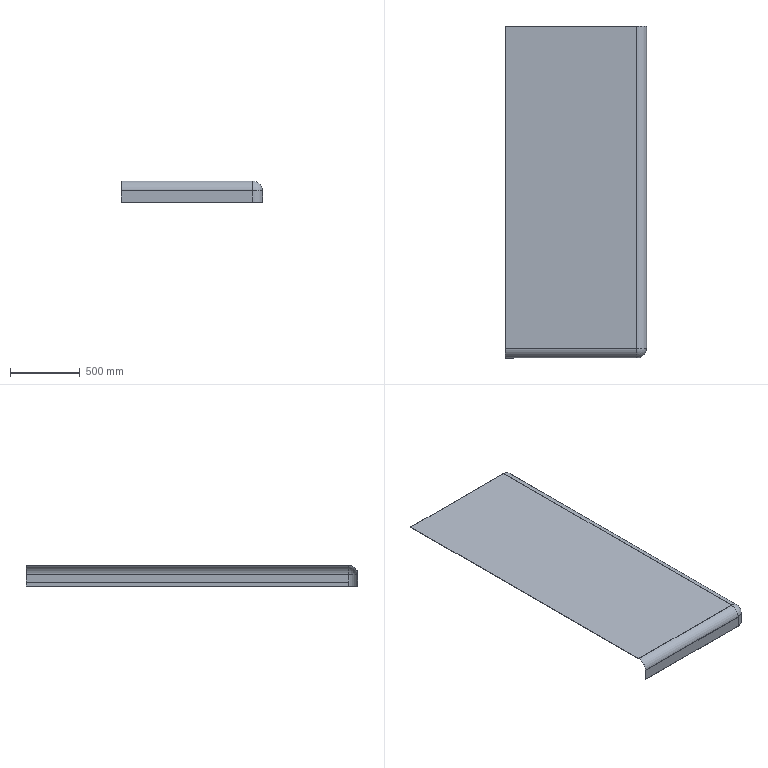Component | SolidWorks | A-SideAluminumCasingAssembly-1_A-SideAluminumCasing3-1 | 1 solid | 38 faces | box 1009.5 x 2375.5 x 154.5 mm | volume 8957048 mm3 | plane 26 | cylinder 10 | torus 2 | commonest cylinder face diameters 139 x2 133 x2 10 x2 4 x2 141 x1 135 x1
STEP:
#1=COLOUR_RGB('',0.7922,0.8196,0.9333);
#2=FILL_AREA_STYLE_COLOUR('',#1);
#3=FILL_AREA_STYLE('',(#2));
#4=SURFACE_STYLE_FILL_AREA(#3);
#5=SURFACE_SIDE_STYLE('',(#4));
#6=SURFACE_STYLE_USAGE(.BOTH.,#5);
#7=PRESENTATION_STYLE_ASSIGNMENT((#6));
#8=CARTESIAN_POINT('',(43.543,0.,73.937));
#9=VERTEX_POINT('',#8);
#10=CARTESIAN_POINT('',(43.543,0.,73.819));
#11=VERTEX_POINT('',#10);
#12=CARTESIAN_POINT('',(43.543,0.,73.819));
#13=DIRECTION('',(0.,-0.,-1.));
#14=VECTOR('',#13,39.37);
#15=LINE('',#12,#14);
#16=EDGE_CURVE('',#9,#11,#15,.T.);
#17=ORIENTED_EDGE('',*,*,#16,.F.);
#18=CARTESIAN_POINT('',(43.543,90.787,73.937));
#19=VERTEX_POINT('',#18);
#20=CARTESIAN_POINT('',(43.543,0.,73.937));
#21=DIRECTION('',(-0.,1.,-0.));
#22=VECTOR('',#21,39.37);
#23=LINE('',#20,#22);
#24=EDGE_CURVE('',#9,#19,#23,.T.);
#25=ORIENTED_EDGE('',*,*,#24,.T.);
#26=CARTESIAN_POINT('',(43.543,90.787,73.819));
#27=VERTEX_POINT('',#26);
#28=CARTESIAN_POINT('',(43.543,90.787,73.819));
#29=DIRECTION('',(0.,-0.,-1.));
#30=VECTOR('',#29,39.37);
#31=LINE('',#28,#30);
#32=EDGE_CURVE('',#19,#27,#31,.T.);
#33=ORIENTED_EDGE('',*,*,#32,.T.);
#34=CARTESIAN_POINT('',(43.543,0.,73.819));
#35=DIRECTION('',(-0.,1.,-0.));
#36=VECTOR('',#35,39.37);
#37=LINE('',#34,#36);
#38=EDGE_CURVE('',#11,#27,#37,.T.);
#39=ORIENTED_EDGE('',*,*,#38,.F.);
#40=EDGE_LOOP('',(#17,#25,#33,#39));
#41=FACE_OUTER_BOUND('',#40,.T.);
#42=CARTESIAN_POINT('',(43.543,0.,73.819));
#43=DIRECTION('',(1.,0.,0.));
#44=DIRECTION('',(-0.,1.,-0.));
#45=AXIS2_PLACEMENT_3D('',#42,#43,#44);
#46=PLANE('',#45);
#47=ADVANCED_FACE('',(#41),#46,.F.);
#48=ORIENTED_EDGE('',*,*,#32,.F.);
#49=CARTESIAN_POINT('',(80.551,90.787,73.937));
#50=VERTEX_POINT('',#49);
#51=CARTESIAN_POINT('',(80.551,90.787,73.937));
#52=DIRECTION('',(1.,0.,0.));
#53=VECTOR('',#52,39.37);
#54=LINE('',#51,#53);
#55=EDGE_CURVE('',#19,#50,#54,.T.);
#56=ORIENTED_EDGE('',*,*,#55,.T.);
#57=CARTESIAN_POINT('',(80.551,90.787,73.819));
#58=VERTEX_POINT('',#57);
#59=CARTESIAN_POINT('',(80.551,90.787,73.819));
#60=DIRECTION('',(0.,-0.,-1.));
#61=VECTOR('',#60,39.37);
#62=LINE('',#59,#61);
#63=EDGE_CURVE('',#50,#58,#62,.T.);
#64=ORIENTED_EDGE('',*,*,#63,.T.);
#65=CARTESIAN_POINT('',(80.551,90.787,73.819));
#66=DIRECTION('',(1.,0.,0.));
#67=VECTOR('',#66,39.37);
#68=LINE('',#65,#67);
#69=EDGE_CURVE('',#27,#58,#68,.T.);
#70=ORIENTED_EDGE('',*,*,#69,.F.);
#71=EDGE_LOOP('',(#48,#56,#64,#70));
#72=FACE_OUTER_BOUND('',#71,.T.);
#73=CARTESIAN_POINT('',(80.551,90.787,73.819));
#74=DIRECTION('',(0.,-1.,0.));
#75=DIRECTION('',(1.,0.,0.));
#76=AXIS2_PLACEMENT_3D('',#73,#74,#75);
#77=PLANE('',#76);
#78=ADVANCED_FACE('',(#72),#77,.F.);
#79=CARTESIAN_POINT('',(80.551,0.03937,73.819));
#80=VERTEX_POINT('',#79);
#81=CARTESIAN_POINT('',(80.551,0.,73.819));
#82=DIRECTION('',(0.,-1.,0.));
#83=VECTOR('',#82,39.37);
#84=LINE('',#81,#83);
#85=EDGE_CURVE('',#58,#80,#84,.T.);
#86=ORIENTED_EDGE('',*,*,#85,.T.);
#87=CARTESIAN_POINT('',(80.512,0.,73.819));
#88=VERTEX_POINT('',#87);
#89=CARTESIAN_POINT('',(80.512,0.03937,73.819));
#90=DIRECTION('',(0.,-0.,-1.));
#91=DIRECTION('',(1.,0.,0.));
#92=AXIS2_PLACEMENT_3D('',#89,#90,#91);
#93=CIRCLE('',#92,0.03937);
#94=EDGE_CURVE('',#80,#88,#93,.T.);
#95=ORIENTED_EDGE('',*,*,#94,.T.);
#96=CARTESIAN_POINT('',(80.551,0.,73.819));
#97=DIRECTION('',(-1.,-0.,-0.));
#98=VECTOR('',#97,39.37);
#99=LINE('',#96,#98);
#100=EDGE_CURVE('',#88,#11,#99,.T.);
#101=ORIENTED_EDGE('',*,*,#100,.T.);
#102=ORIENTED_EDGE('',*,*,#38,.T.);
#103=ORIENTED_EDGE('',*,*,#69,.T.);
#104=EDGE_LOOP('',(#86,#95,#101,#102,#103));
#105=FACE_OUTER_BOUND('',#104,.T.);
#106=CARTESIAN_POINT('',(80.551,0.,73.819));
#107=DIRECTION('',(-0.,0.,1.));
#108=DIRECTION('',(1.,0.,0.));
#109=AXIS2_PLACEMENT_3D('',#106,#107,#108);
#110=PLANE('',#109);
#111=ADVANCED_FACE('',(#105),#110,.F.);
#112=CARTESIAN_POINT('',(80.512,0.,73.937));
#113=VERTEX_POINT('',#112);
#114=CARTESIAN_POINT('',(80.551,0.,73.937));
#115=DIRECTION('',(-1.,-0.,-0.));
#116=VECTOR('',#115,39.37);
#117=LINE('',#114,#116);
#118=EDGE_CURVE('',#113,#9,#117,.T.);
#119=ORIENTED_EDGE('',*,*,#118,.F.);
#120=CARTESIAN_POINT('',(80.551,0.03937,73.937));
#121=VERTEX_POINT('',#120);
#122=CARTESIAN_POINT('',(80.512,0.03937,73.937));
#123=DIRECTION('',(-0.,0.,1.));
#124=DIRECTION('',(1.,0.,0.));
#125=AXIS2_PLACEMENT_3D('',#122,#123,#124);
#126=CIRCLE('',#125,0.03937);
#127=EDGE_CURVE('',#113,#121,#126,.T.);
#128=ORIENTED_EDGE('',*,*,#127,.T.);
#129=CARTESIAN_POINT('',(80.551,0.,73.937));
#130=DIRECTION('',(0.,-1.,0.));
#131=VECTOR('',#130,39.37);
#132=LINE('',#129,#131);
#133=EDGE_CURVE('',#50,#121,#132,.T.);
#134=ORIENTED_EDGE('',*,*,#133,.F.);
#135=ORIENTED_EDGE('',*,*,#55,.F.);
#136=ORIENTED_EDGE('',*,*,#24,.F.);
#137=EDGE_LOOP('',(#119,#128,#134,#135,#136));
#138=FACE_OUTER_BOUND('',#137,.T.);
#139=CARTESIAN_POINT('',(80.551,0.,73.937));
#140=DIRECTION('',(-0.,0.,1.));
#141=DIRECTION('',(1.,0.,0.));
#142=AXIS2_PLACEMENT_3D('',#139,#140,#141);
#143=PLANE('',#142);
#144=ADVANCED_FACE('',(#138),#143,.T.);
#145=CARTESIAN_POINT('',(43.543,-2.618,71.201));
#146=VERTEX_POINT('',#145);
#147=CARTESIAN_POINT('',(43.543,0.,71.201));
#148=DIRECTION('',(-1.,-0.,-0.));
#149=DIRECTION('',(0.,0.,1.));
#150=AXIS2_PLACEMENT_3D('',#147,#148,#149);
#151=CIRCLE('',#150,2.618);
#152=EDGE_CURVE('',#146,#11,#151,.T.);
#153=ORIENTED_EDGE('',*,*,#152,.F.);
#154=CARTESIAN_POINT('',(43.543,-2.736,71.201));
#155=VERTEX_POINT('',#154);
#156=CARTESIAN_POINT('',(43.543,-2.618,71.201));
#157=DIRECTION('',(0.,-1.,0.));
#158=VECTOR('',#157,39.37);
#159=LINE('',#156,#158);
#160=EDGE_CURVE('',#146,#155,#159,.T.);
#161=ORIENTED_EDGE('',*,*,#160,.T.);
#162=CARTESIAN_POINT('',(43.543,0.,71.201));
#163=DIRECTION('',(-1.,-0.,-0.));
#164=DIRECTION('',(0.,0.,1.));
#165=AXIS2_PLACEMENT_3D('',#162,#163,#164);
#166=CIRCLE('',#165,2.736);
#167=EDGE_CURVE('',#155,#9,#166,.T.);
#168=ORIENTED_EDGE('',*,*,#167,.T.);
#169=ORIENTED_EDGE('',*,*,#16,.T.);
#170=EDGE_LOOP('',(#153,#161,#168,#169));
#171=FACE_OUTER_BOUND('',#170,.T.);
#172=CARTESIAN_POINT('',(43.543,0.,71.201));
#173=DIRECTION('',(1.,0.,0.));
#174=DIRECTION('',(0.,-0.,-1.));
#175=AXIS2_PLACEMENT_3D('',#172,#173,#174);
#176=PLANE('',#175);
#177=ADVANCED_FACE('',(#171),#176,.F.);
#178=ORIENTED_EDGE('',*,*,#118,.T.);
#179=ORIENTED_EDGE('',*,*,#167,.F.);
#180=CARTESIAN_POINT('',(80.512,-2.736,71.201));
#181=VERTEX_POINT('',#180);
#182=CARTESIAN_POINT('',(80.512,-2.736,71.201));
#183=DIRECTION('',(1.,0.,0.));
#184=VECTOR('',#183,39.37);
#185=LINE('',#182,#184);
#186=EDGE_CURVE('',#155,#181,#185,.T.);
#187=ORIENTED_EDGE('',*,*,#186,.T.);
#188=CARTESIAN_POINT('',(80.512,0.,71.201));
#189=DIRECTION('',(1.,0.,0.));
#190=DIRECTION('',(0.,0.,1.));
#191=AXIS2_PLACEMENT_3D('',#188,#189,#190);
#192=CIRCLE('',#191,2.736);
#193=EDGE_CURVE('',#113,#181,#192,.T.);
#194=ORIENTED_EDGE('',*,*,#193,.F.);
#195=EDGE_LOOP('',(#178,#179,#187,#194));
#196=FACE_OUTER_BOUND('',#195,.T.);
#197=CARTESIAN_POINT('',(43.543,0.,71.201));
#198=DIRECTION('',(-1.,-0.,-0.));
#199=DIRECTION('',(0.,-1.,0.));
#200=AXIS2_PLACEMENT_3D('',#197,#198,#199);
#201=CYLINDRICAL_SURFACE('',#200,2.736);
#202=ADVANCED_FACE('',(#196),#201,.T.);
#203=ORIENTED_EDGE('',*,*,#100,.F.);
#204=CARTESIAN_POINT('',(80.512,-2.618,71.201));
#205=VERTEX_POINT('',#204);
#206=CARTESIAN_POINT('',(80.512,0.,71.201));
#207=DIRECTION('',(1.,0.,0.));
#208=DIRECTION('',(0.,0.,1.));
#209=AXIS2_PLACEMENT_3D('',#206,#207,#208);
#210=CIRCLE('',#209,2.618);
#211=EDGE_CURVE('',#88,#205,#210,.T.);
#212=ORIENTED_EDGE('',*,*,#211,.T.);
#213=CARTESIAN_POINT('',(80.512,-2.618,71.201));
#214=DIRECTION('',(-1.,-0.,-0.));
#215=VECTOR('',#214,39.37);
#216=LINE('',#213,#215);
#217=EDGE_CURVE('',#205,#146,#216,.T.);
#218=ORIENTED_EDGE('',*,*,#217,.T.);
#219=ORIENTED_EDGE('',*,*,#152,.T.);
#220=EDGE_LOOP('',(#203,#212,#218,#219));
#221=FACE_OUTER_BOUND('',#220,.T.);
#222=CARTESIAN_POINT('',(43.543,0.,71.201));
#223=DIRECTION('',(-1.,-0.,-0.));
#224=DIRECTION('',(0.,-1.,0.));
#225=AXIS2_PLACEMENT_3D('',#222,#223,#224);
#226=CYLINDRICAL_SURFACE('',#225,2.618);
#227=ADVANCED_FACE('',(#221),#226,.F.);
#228=ORIENTED_EDGE('',*,*,#160,.F.);
#229=CARTESIAN_POINT('',(43.543,-2.618,68.051));
#230=VERTEX_POINT('',#229);
#231=CARTESIAN_POINT('',(43.543,-2.618,68.051));
#232=DIRECTION('',(0.,-0.,-1.));
#233=VECTOR('',#232,39.37);
#234=LINE('',#231,#233);
#235=EDGE_CURVE('',#146,#230,#234,.T.);
#236=ORIENTED_EDGE('',*,*,#235,.T.);
#237=CARTESIAN_POINT('',(43.543,-2.736,68.051));
#238=VERTEX_POINT('',#237);
#239=CARTESIAN_POINT('',(43.543,-2.736,68.051));
#240=DIRECTION('',(-0.,1.,-0.));
#241=VECTOR('',#240,39.37);
#242=LINE('',#239,#241);
#243=EDGE_CURVE('',#238,#230,#242,.T.);
#244=ORIENTED_EDGE('',*,*,#243,.F.);
#245=CARTESIAN_POINT('',(43.543,-2.736,73.819));
#246=DIRECTION('',(0.,-0.,-1.));
#247=VECTOR('',#246,39.37);
#248=LINE('',#245,#247);
#249=EDGE_CURVE('',#155,#238,#248,.T.);
#250=ORIENTED_EDGE('',*,*,#249,.F.);
#251=EDGE_LOOP('',(#228,#236,#244,#250));
#252=FACE_OUTER_BOUND('',#251,.T.);
#253=CARTESIAN_POINT('',(43.543,-2.736,68.051));
#254=DIRECTION('',(1.,0.,0.));
#255=DIRECTION('',(0.,-0.,-1.));
#256=AXIS2_PLACEMENT_3D('',#253,#254,#255);
#257=PLANE('',#256);
#258=ADVANCED_FACE('',(#252),#257,.F.);
#259=ORIENTED_EDGE('',*,*,#186,.F.);
#260=ORIENTED_EDGE('',*,*,#249,.T.);
#261=CARTESIAN_POINT('',(80.512,-2.736,68.051));
#262=VERTEX_POINT('',#261);
#263=CARTESIAN_POINT('',(80.551,-2.736,68.051));
#264=DIRECTION('',(1.,0.,0.));
#265=VECTOR('',#264,39.37);
#266=LINE('',#263,#265);
#267=EDGE_CURVE('',#238,#262,#266,.T.);
#268=ORIENTED_EDGE('',*,*,#267,.T.);
#269=CARTESIAN_POINT('',(80.512,-2.736,73.819));
#270=DIRECTION('',(-0.,0.,1.));
#271=VECTOR('',#270,39.37);
#272=LINE('',#269,#271);
#273=EDGE_CURVE('',#262,#181,#272,.T.);
#274=ORIENTED_EDGE('',*,*,#273,.T.);
#275=EDGE_LOOP('',(#259,#260,#268,#274));
#276=FACE_OUTER_BOUND('',#275,.T.);
#277=CARTESIAN_POINT('',(80.551,-2.736,73.819));
#278=DIRECTION('',(-0.,1.,-0.));
#279=DIRECTION('',(0.,-0.,-1.));
#280=AXIS2_PLACEMENT_3D('',#277,#278,#279);
#281=PLANE('',#280);
#282=ADVANCED_FACE('',(#276),#281,.F.);
#283=ORIENTED_EDGE('',*,*,#235,.F.);
#284=ORIENTED_EDGE('',*,*,#217,.F.);
#285=CARTESIAN_POINT('',(80.512,-2.618,68.051));
#286=VERTEX_POINT('',#285);
#287=CARTESIAN_POINT('',(80.512,-2.618,73.819));
#288=DIRECTION('',(-0.,0.,1.));
#289=VECTOR('',#288,39.37);
#290=LINE('',#287,#289);
#291=EDGE_CURVE('',#286,#205,#290,.T.);
#292=ORIENTED_EDGE('',*,*,#291,.F.);
#293=CARTESIAN_POINT('',(80.512,-2.618,68.051));
#294=DIRECTION('',(1.,0.,0.));
#295=VECTOR('',#294,39.37);
#296=LINE('',#293,#295);
#297=EDGE_CURVE('',#230,#286,#296,.T.);
#298=ORIENTED_EDGE('',*,*,#297,.F.);
#299=EDGE_LOOP('',(#283,#284,#292,#298));
#300=FACE_OUTER_BOUND('',#299,.T.);
#301=CARTESIAN_POINT('',(80.551,-2.618,73.819));
#302=DIRECTION('',(-0.,1.,-0.));
#303=DIRECTION('',(0.,-0.,-1.));
#304=AXIS2_PLACEMENT_3D('',#301,#302,#303);
#305=PLANE('',#304);
#306=ADVANCED_FACE('',(#300),#305,.T.);
#307=CARTESIAN_POINT('',(83.169,0.03937,68.051));
#308=VERTEX_POINT('',#307);
#309=CARTESIAN_POINT('',(80.512,0.03937,68.051));
#310=DIRECTION('',(0.,-0.,-1.));
#311=DIRECTION('',(1.,0.,0.));
#312=AXIS2_PLACEMENT_3D('',#309,#310,#311);
#313=CIRCLE('',#312,2.657);
#314=EDGE_CURVE('',#308,#286,#313,.T.);
#315=ORIENTED_EDGE('',*,*,#314,.F.);
#316=CARTESIAN_POINT('',(83.287,0.03937,68.051));
#317=VERTEX_POINT('',#316);
#318=CARTESIAN_POINT('',(83.169,0.03937,68.051));
#319=DIRECTION('',(1.,0.,0.));
#320=VECTOR('',#319,39.37);
#321=LINE('',#318,#320);
#322=EDGE_CURVE('',#308,#317,#321,.T.);
#323=ORIENTED_EDGE('',*,*,#322,.T.);
#324=CARTESIAN_POINT('',(80.512,0.03937,68.051));
#325=DIRECTION('',(0.,-0.,-1.));
#326=DIRECTION('',(1.,0.,0.));
#327=AXIS2_PLACEMENT_3D('',#324,#325,#326);
#328=CIRCLE('',#327,2.776);
#329=EDGE_CURVE('',#317,#262,#328,.T.);
#330=ORIENTED_EDGE('',*,*,#329,.T.);
#331=ORIENTED_EDGE('',*,*,#267,.F.);
#332=ORIENTED_EDGE('',*,*,#243,.T.);
#333=ORIENTED_EDGE('',*,*,#297,.T.);
#334=EDGE_LOOP('',(#315,#323,#330,#331,#332,#333));
#335=FACE_OUTER_BOUND('',#334,.T.);
#336=CARTESIAN_POINT('',(80.512,-2.736,68.051));
#337=DIRECTION('',(-0.,0.,1.));
#338=DIRECTION('',(-0.,1.,-0.));
#339=AXIS2_PLACEMENT_3D('',#336,#337,#338);
#340=PLANE('',#339);
#341=ADVANCED_FACE('',(#335),#340,.F.);
#342=CARTESIAN_POINT('',(83.169,90.787,71.201));
#343=VERTEX_POINT('',#342);
#344=CARTESIAN_POINT('',(83.287,90.787,71.201));
#345=VERTEX_POINT('',#344);
#346=CARTESIAN_POINT('',(83.287,90.787,71.201));
#347=DIRECTION('',(1.,0.,0.));
#348=VECTOR('',#347,39.37);
#349=LINE('',#346,#348);
#350=EDGE_CURVE('',#343,#345,#349,.T.);
#351=ORIENTED_EDGE('',*,*,#350,.F.);
#352=CARTESIAN_POINT('',(80.551,90.787,71.201));
#353=DIRECTION('',(-0.,1.,-0.));
#354=DIRECTION('',(0.,0.,1.));
#355=AXIS2_PLACEMENT_3D('',#352,#353,#354);
#356=CIRCLE('',#355,2.618);
#357=EDGE_CURVE('',#58,#343,#356,.T.);
#358=ORIENTED_EDGE('',*,*,#357,.F.);
#359=ORIENTED_EDGE('',*,*,#63,.F.);
#360=CARTESIAN_POINT('',(80.551,90.787,71.201));
#361=DIRECTION('',(-0.,1.,-0.));
#362=DIRECTION('',(0.,0.,1.));
#363=AXIS2_PLACEMENT_3D('',#360,#361,#362);
#364=CIRCLE('',#363,2.736);
#365=EDGE_CURVE('',#50,#345,#364,.T.);
#366=ORIENTED_EDGE('',*,*,#365,.T.);
#367=EDGE_LOOP('',(#351,#358,#359,#366));
#368=FACE_OUTER_BOUND('',#367,.T.);
#369=CARTESIAN_POINT('',(80.551,90.787,71.201));
#370=DIRECTION('',(-0.,1.,-0.));
#371=DIRECTION('',(0.,-0.,-1.));
#372=AXIS2_PLACEMENT_3D('',#369,#370,#371);
#373=PLANE('',#372);
#374=ADVANCED_FACE('',(#368),#373,.T.);
#375=ORIENTED_EDGE('',*,*,#133,.T.);
#376=CARTESIAN_POINT('',(83.287,0.03937,71.201));
#377=VERTEX_POINT('',#376);
#378=CARTESIAN_POINT('',(80.551,0.03937,71.201));
#379=DIRECTION('',(0.,-1.,0.));
#380=DIRECTION('',(0.,0.,1.));
#381=AXIS2_PLACEMENT_3D('',#378,#379,#380);
#382=CIRCLE('',#381,2.736);
#383=EDGE_CURVE('',#377,#121,#382,.T.);
#384=ORIENTED_EDGE('',*,*,#383,.F.);
#385=CARTESIAN_POINT('',(83.287,90.787,71.201));
#386=DIRECTION('',(-0.,1.,-0.));
#387=VECTOR('',#386,39.37);
#388=LINE('',#385,#387);
#389=EDGE_CURVE('',#377,#345,#388,.T.);
#390=ORIENTED_EDGE('',*,*,#389,.T.);
#391=ORIENTED_EDGE('',*,*,#365,.F.);
#392=EDGE_LOOP('',(#375,#384,#390,#391));
#393=FACE_OUTER_BOUND('',#392,.T.);
#394=CARTESIAN_POINT('',(80.551,0.03937,71.201));
#395=DIRECTION('',(0.,-1.,0.));
#396=DIRECTION('',(1.,0.,0.));
#397=AXIS2_PLACEMENT_3D('',#394,#395,#396);
#398=CYLINDRICAL_SURFACE('',#397,2.736);
#399=ADVANCED_FACE('',(#393),#398,.T.);
#400=ORIENTED_EDGE('',*,*,#85,.F.);
#401=ORIENTED_EDGE('',*,*,#357,.T.);
#402=CARTESIAN_POINT('',(83.169,0.03937,71.201));
#403=VERTEX_POINT('',#402);
#404=CARTESIAN_POINT('',(83.169,90.787,71.201));
#405=DIRECTION('',(0.,-1.,0.));
#406=VECTOR('',#405,39.37);
#407=LINE('',#404,#406);
#408=EDGE_CURVE('',#343,#403,#407,.T.);
#409=ORIENTED_EDGE('',*,*,#408,.T.);
#410=CARTESIAN_POINT('',(80.551,0.03937,71.201));
#411=DIRECTION('',(0.,-1.,0.));
#412=DIRECTION('',(0.,0.,1.));
#413=AXIS2_PLACEMENT_3D('',#410,#411,#412);
#414=CIRCLE('',#413,2.618);
#415=EDGE_CURVE('',#403,#80,#414,.T.);
#416=ORIENTED_EDGE('',*,*,#415,.T.);
#417=EDGE_LOOP('',(#400,#401,#409,#416));
#418=FACE_OUTER_BOUND('',#417,.T.);
#419=CARTESIAN_POINT('',(80.551,0.03937,71.201));
#420=DIRECTION('',(0.,-1.,0.));
#421=DIRECTION('',(1.,0.,0.));
#422=AXIS2_PLACEMENT_3D('',#419,#420,#421);
#423=CYLINDRICAL_SURFACE('',#422,2.618);
#424=ADVANCED_FACE('',(#418),#423,.F.);
#425=ORIENTED_EDGE('',*,*,#350,.T.);
#426=CARTESIAN_POINT('',(83.287,90.787,68.051));
#427=VERTEX_POINT('',#426);
#428=CARTESIAN_POINT('',(83.287,90.787,73.819));
#429=DIRECTION('',(-0.,0.,1.));
#430=VECTOR('',#429,39.37);
#431=LINE('',#428,#430);
#432=EDGE_CURVE('',#427,#345,#431,.T.);
#433=ORIENTED_EDGE('',*,*,#432,.F.);
#434=CARTESIAN_POINT('',(83.169,90.787,68.051));
#435=VERTEX_POINT('',#434);
#436=CARTESIAN_POINT('',(83.287,90.787,68.051));
#437=DIRECTION('',(-1.,-0.,-0.));
#438=VECTOR('',#437,39.37);
#439=LINE('',#436,#438);
#440=EDGE_CURVE('',#427,#435,#439,.T.);
#441=ORIENTED_EDGE('',*,*,#440,.T.);
#442=CARTESIAN_POINT('',(83.169,90.787,73.819));
#443=DIRECTION('',(-0.,0.,1.));
#444=VECTOR('',#443,39.37);
#445=LINE('',#442,#444);
#446=EDGE_CURVE('',#435,#343,#445,.T.);
#447=ORIENTED_EDGE('',*,*,#446,.T.);
#448=EDGE_LOOP('',(#425,#433,#441,#447));
#449=FACE_OUTER_BOUND('',#448,.T.);
#450=CARTESIAN_POINT('',(83.287,90.787,73.819));
#451=DIRECTION('',(0.,-1.,0.));
#452=DIRECTION('',(-0.,0.,1.));
#453=AXIS2_PLACEMENT_3D('',#450,#451,#452);
#454=PLANE('',#453);
#455=ADVANCED_FACE('',(#449),#454,.F.);
#456=ORIENTED_EDGE('',*,*,#389,.F.);
#457=CARTESIAN_POINT('',(83.287,0.03937,73.819));
#458=DIRECTION('',(0.,-0.,-1.));
#459=VECTOR('',#458,39.37);
#460=LINE('',#457,#459);
#461=EDGE_CURVE('',#377,#317,#460,.T.);
#462=ORIENTED_EDGE('',*,*,#461,.T.);
#463=CARTESIAN_POINT('',(83.287,0.,68.051));
#464=DIRECTION('',(-0.,1.,-0.));
#465=VECTOR('',#464,39.37);
#466=LINE('',#463,#465);
#467=EDGE_CURVE('',#317,#427,#466,.T.);
#468=ORIENTED_EDGE('',*,*,#467,.T.);
#469=ORIENTED_EDGE('',*,*,#432,.T.);
#470=EDGE_LOOP('',(#456,#462,#468,#469));
#471=FACE_OUTER_BOUND('',#470,.T.);
#472=CARTESIAN_POINT('',(83.287,0.,73.819));
#473=DIRECTION('',(-1.,-0.,-0.));
#474=DIRECTION('',(-0.,0.,1.));
#475=AXIS2_PLACEMENT_3D('',#472,#473,#474);
#476=PLANE('',#475);
#477=ADVANCED_FACE('',(#471),#476,.F.);
#478=CARTESIAN_POINT('',(83.169,0.03937,68.051));
#479=DIRECTION('',(0.,-0.,-1.));
#480=VECTOR('',#479,39.37);
#481=LINE('',#478,#480);
#482=EDGE_CURVE('',#403,#308,#481,.T.);
#483=ORIENTED_EDGE('',*,*,#482,.F.);
#484=ORIENTED_EDGE('',*,*,#408,.F.);
#485=ORIENTED_EDGE('',*,*,#446,.F.);
#486=CARTESIAN_POINT('',(83.169,90.787,68.051));
#487=DIRECTION('',(-0.,1.,-0.));
#488=VECTOR('',#487,39.37);
#489=LINE('',#486,#488);
#490=EDGE_CURVE('',#308,#435,#489,.T.);
#491=ORIENTED_EDGE('',*,*,#490,.F.);
#492=EDGE_LOOP('',(#483,#484,#485,#491));
#493=FACE_OUTER_BOUND('',#492,.T.);
#494=CARTESIAN_POINT('',(83.169,0.,73.819));
#495=DIRECTION('',(-1.,-0.,-0.));
#496=DIRECTION('',(-0.,0.,1.));
#497=AXIS2_PLACEMENT_3D('',#494,#495,#496);
#498=PLANE('',#497);
#499=ADVANCED_FACE('',(#493),#498,.T.);
#500=ORIENTED_EDGE('',*,*,#94,.F.);
#501=ORIENTED_EDGE('',*,*,#415,.F.);
#502=CARTESIAN_POINT('',(80.512,0.03937,71.201));
#503=DIRECTION('',(0.,-0.,-1.));
#504=DIRECTION('',(1.,0.,0.));
#505=AXIS2_PLACEMENT_3D('',#502,#503,#504);
#506=CIRCLE('',#505,2.657);
#507=EDGE_CURVE('',#403,#205,#506,.T.);
#508=ORIENTED_EDGE('',*,*,#507,.T.);
#509=ORIENTED_EDGE('',*,*,#211,.F.);
#510=EDGE_LOOP('',(#500,#501,#508,#509));
#511=FACE_OUTER_BOUND('',#510,.T.);
#512=CARTESIAN_POINT('',(80.512,0.03937,71.201));
#513=DIRECTION('',(0.,-0.,-1.));
#514=DIRECTION('',(-1.,-0.,-0.));
#515=AXIS2_PLACEMENT_3D('',#512,#513,#514);
#516=TOROIDAL_SURFACE('',#515,0.03937,2.618);
#517=ADVANCED_FACE('',(#511),#516,.F.);
#518=CARTESIAN_POINT('',(80.512,0.03937,71.201));
#519=DIRECTION('',(0.,-0.,-1.));
#520=DIRECTION('',(1.,0.,0.));
#521=AXIS2_PLACEMENT_3D('',#518,#519,#520);
#522=CIRCLE('',#521,2.776);
#523=EDGE_CURVE('',#377,#181,#522,.T.);
#524=ORIENTED_EDGE('',*,*,#523,.F.);
#525=ORIENTED_EDGE('',*,*,#383,.T.);
#526=ORIENTED_EDGE('',*,*,#127,.F.);
#527=ORIENTED_EDGE('',*,*,#193,.T.);
#528=EDGE_LOOP('',(#524,#525,#526,#527));
#529=FACE_OUTER_BOUND('',#528,.T.);
#530=CARTESIAN_POINT('',(80.512,0.03937,71.201));
#531=DIRECTION('',(0.,-0.,-1.));
#532=DIRECTION('',(-1.,-0.,-0.));
#533=AXIS2_PLACEMENT_3D('',#530,#531,#532);
#534=TOROIDAL_SURFACE('',#533,0.03937,2.736);
#535=ADVANCED_FACE('',(#529),#534,.T.);
#536=ORIENTED_EDGE('',*,*,#329,.F.);
#537=ORIENTED_EDGE('',*,*,#461,.F.);
#538=ORIENTED_EDGE('',*,*,#523,.T.);
#539=ORIENTED_EDGE('',*,*,#273,.F.);
#540=EDGE_LOOP('',(#536,#537,#538,#539));
#541=FACE_OUTER_BOUND('',#540,.T.);
#542=CARTESIAN_POINT('',(80.512,0.03937,71.201));
#543=DIRECTION('',(0.,-0.,-1.));
#544=DIRECTION('',(-1.,-0.,0.));
#545=AXIS2_PLACEMENT_3D('',#542,#543,#544);
#546=CYLINDRICAL_SURFACE('',#545,2.776);
#547=ADVANCED_FACE('',(#541),#546,.T.);
#548=ORIENTED_EDGE('',*,*,#507,.F.);
#549=ORIENTED_EDGE('',*,*,#482,.T.);
#550=ORIENTED_EDGE('',*,*,#314,.T.);
#551=ORIENTED_EDGE('',*,*,#291,.T.);
#552=EDGE_LOOP('',(#548,#549,#550,#551));
#553=FACE_OUTER_BOUND('',#552,.T.);
#554=CARTESIAN_POINT('',(80.512,0.03937,71.201));
#555=DIRECTION('',(0.,-0.,-1.));
#556=DIRECTION('',(-1.,-0.,0.));
#557=AXIS2_PLACEMENT_3D('',#554,#555,#556);
#558=CYLINDRICAL_SURFACE('',#557,2.657);
#559=ADVANCED_FACE('',(#553),#558,.F.);
#560=CARTESIAN_POINT('',(83.091,90.787,67.972));
#561=VERTEX_POINT('',#560);
#562=CARTESIAN_POINT('',(83.091,90.787,67.854));
#563=VERTEX_POINT('',#562);
#564=CARTESIAN_POINT('',(83.091,90.787,67.972));
#565=DIRECTION('',(0.,-0.,-1.));
#566=VECTOR('',#565,39.37);
#567=LINE('',#564,#566);
#568=EDGE_CURVE('',#561,#563,#567,.T.);
#569=ORIENTED_EDGE('',*,*,#568,.T.);
#570=CARTESIAN_POINT('',(81.28,90.787,67.854));
#571=VERTEX_POINT('',#570);
#572=CARTESIAN_POINT('',(81.28,90.787,67.854));
#573=DIRECTION('',(1.,0.,0.));
#574=VECTOR('',#573,39.37);
#575=LINE('',#572,#574);
#576=EDGE_CURVE('',#571,#563,#575,.T.);
#577=ORIENTED_EDGE('',*,*,#576,.F.);
#578=CARTESIAN_POINT('',(81.28,90.787,67.972));
#579=VERTEX_POINT('',#578);
#580=CARTESIAN_POINT('',(81.28,90.787,67.972));
#581=DIRECTION('',(0.,-0.,-1.));
#582=VECTOR('',#581,39.37);
#583=LINE('',#580,#582);
#584=EDGE_CURVE('',#579,#571,#583,.T.);
#585=ORIENTED_EDGE('',*,*,#584,.F.);
#586=CARTESIAN_POINT('',(81.28,90.787,67.972));
#587=DIRECTION('',(1.,0.,0.));
#588=VECTOR('',#587,39.37);
#589=LINE('',#586,#588);
#590=EDGE_CURVE('',#579,#561,#589,.T.);
#591=ORIENTED_EDGE('',*,*,#590,.T.);
#592=EDGE_LOOP('',(#569,#577,#585,#591));
#593=FACE_OUTER_BOUND('',#592,.T.);
#594=CARTESIAN_POINT('',(81.28,90.787,67.972));
#595=DIRECTION('',(-0.,1.,-0.));
#596=DIRECTION('',(1.,0.,0.));
#597=AXIS2_PLACEMENT_3D('',#594,#595,#596);
#598=PLANE('',#597);
#599=ADVANCED_FACE('',(#593),#598,.T.);
#600=ORIENTED_EDGE('',*,*,#584,.T.);
#601=CARTESIAN_POINT('',(81.083,90.787,68.051));
#602=VERTEX_POINT('',#601);
#603=CARTESIAN_POINT('',(81.28,90.787,68.051));
#604=DIRECTION('',(-0.,1.,-0.));
#605=DIRECTION('',(0.,0.,1.));
#606=AXIS2_PLACEMENT_3D('',#603,#604,#605);
#607=CIRCLE('',#606,0.1969);
#608=EDGE_CURVE('',#571,#602,#607,.T.);
#609=ORIENTED_EDGE('',*,*,#608,.T.);
#610=CARTESIAN_POINT('',(81.201,90.787,68.051));
#611=VERTEX_POINT('',#610);
#612=CARTESIAN_POINT('',(81.201,90.787,68.051));
#613=DIRECTION('',(-1.,-0.,-0.));
#614=VECTOR('',#613,39.37);
#615=LINE('',#612,#614);
#616=EDGE_CURVE('',#611,#602,#615,.T.);
#617=ORIENTED_EDGE('',*,*,#616,.F.);
#618=CARTESIAN_POINT('',(81.28,90.787,68.051));
#619=DIRECTION('',(-0.,1.,-0.));
#620=DIRECTION('',(0.,0.,1.));
#621=AXIS2_PLACEMENT_3D('',#618,#619,#620);
#622=CIRCLE('',#621,0.07874);
#623=EDGE_CURVE('',#579,#611,#622,.T.);
#624=ORIENTED_EDGE('',*,*,#623,.F.);
#625=EDGE_LOOP('',(#600,#609,#617,#624));
#626=FACE_OUTER_BOUND('',#625,.T.);
#627=CARTESIAN_POINT('',(81.28,90.787,68.051));
#628=DIRECTION('',(-0.,1.,-0.));
#629=DIRECTION('',(0.,-0.,-1.));
#630=AXIS2_PLACEMENT_3D('',#627,#628,#629);
#631=PLANE('',#630);
#632=ADVANCED_FACE('',(#626),#631,.T.);
#633=ORIENTED_EDGE('',*,*,#616,.T.);
#634=CARTESIAN_POINT('',(81.083,90.787,69.154));
#635=VERTEX_POINT('',#634);
#636=CARTESIAN_POINT('',(81.083,90.787,67.972));
#637=DIRECTION('',(-0.,0.,1.));
#638=VECTOR('',#637,39.37);
#639=LINE('',#636,#638);
#640=EDGE_CURVE('',#602,#635,#639,.T.);
#641=ORIENTED_EDGE('',*,*,#640,.T.);
#642=CARTESIAN_POINT('',(81.201,90.787,69.154));
#643=VERTEX_POINT('',#642);
#644=CARTESIAN_POINT('',(81.201,90.787,69.154));
#645=DIRECTION('',(-1.,-0.,-0.));
#646=VECTOR('',#645,39.37);
#647=LINE('',#644,#646);
#648=EDGE_CURVE('',#643,#635,#647,.T.);
#649=ORIENTED_EDGE('',*,*,#648,.F.);
#650=CARTESIAN_POINT('',(81.201,90.787,67.972));
#651=DIRECTION('',(-0.,0.,1.));
#652=VECTOR('',#651,39.37);
#653=LINE('',#650,#652);
#654=EDGE_CURVE('',#611,#643,#653,.T.);
#655=ORIENTED_EDGE('',*,*,#654,.F.);
#656=EDGE_LOOP('',(#633,#641,#649,#655));
#657=FACE_OUTER_BOUND('',#656,.T.);
#658=CARTESIAN_POINT('',(81.201,90.787,67.972));
#659=DIRECTION('',(-0.,1.,-0.));
#660=DIRECTION('',(-0.,0.,1.));
#661=AXIS2_PLACEMENT_3D('',#658,#659,#660);
#662=PLANE('',#661);
#663=ADVANCED_FACE('',(#657),#662,.T.);
#664=ORIENTED_EDGE('',*,*,#648,.T.);
#665=CARTESIAN_POINT('',(81.083,0.03937,69.154));
#666=VERTEX_POINT('',#665);
#667=CARTESIAN_POINT('',(81.083,90.787,69.154));
#668=DIRECTION('',(0.,-1.,0.));
#669=VECTOR('',#668,39.37);
#670=LINE('',#667,#669);
#671=EDGE_CURVE('',#635,#666,#670,.T.);
#672=ORIENTED_EDGE('',*,*,#671,.T.);
#673=CARTESIAN_POINT('',(81.201,0.03937,69.154));
#674=VERTEX_POINT('',#673);
#675=CARTESIAN_POINT('',(81.201,0.03937,69.154));
#676=DIRECTION('',(-1.,-0.,-0.));
#677=VECTOR('',#676,39.37);
#678=LINE('',#675,#677);
#679=EDGE_CURVE('',#674,#666,#678,.T.);
#680=ORIENTED_EDGE('',*,*,#679,.F.);
#681=CARTESIAN_POINT('',(81.201,90.787,69.154));
#682=DIRECTION('',(0.,-1.,0.));
#683=VECTOR('',#682,39.37);
#684=LINE('',#681,#683);
#685=EDGE_CURVE('',#643,#674,#684,.T.);
#686=ORIENTED_EDGE('',*,*,#685,.F.);
#687=EDGE_LOOP('',(#664,#672,#680,#686));
#688=FACE_OUTER_BOUND('',#687,.T.);
#689=CARTESIAN_POINT('',(81.201,90.787,69.154));
#690=DIRECTION('',(-0.,0.,1.));
#691=DIRECTION('',(0.,-1.,0.));
#692=AXIS2_PLACEMENT_3D('',#689,#690,#691);
#693=PLANE('',#692);
#694=ADVANCED_FACE('',(#688),#693,.T.);
#695=ORIENTED_EDGE('',*,*,#679,.T.);
#696=CARTESIAN_POINT('',(81.083,0.03937,68.051));
#697=VERTEX_POINT('',#696);
#698=CARTESIAN_POINT('',(81.083,0.03937,67.972));
#699=DIRECTION('',(0.,-0.,-1.));
#700=VECTOR('',#699,39.37);
#701=LINE('',#698,#700);
#702=EDGE_CURVE('',#666,#697,#701,.T.);
#703=ORIENTED_EDGE('',*,*,#702,.T.);
#704=CARTESIAN_POINT('',(81.201,0.03937,68.051));
#705=VERTEX_POINT('',#704);
#706=CARTESIAN_POINT('',(81.201,0.03937,68.051));
#707=DIRECTION('',(-1.,-0.,-0.));
#708=VECTOR('',#707,39.37);
#709=LINE('',#706,#708);
#710=EDGE_CURVE('',#705,#697,#709,.T.);
#711=ORIENTED_EDGE('',*,*,#710,.F.);
#712=CARTESIAN_POINT('',(81.201,0.03937,67.972));
#713=DIRECTION('',(0.,-0.,-1.));
#714=VECTOR('',#713,39.37);
#715=LINE('',#712,#714);
#716=EDGE_CURVE('',#674,#705,#715,.T.);
#717=ORIENTED_EDGE('',*,*,#716,.F.);
#718=EDGE_LOOP('',(#695,#703,#711,#717));
#719=FACE_OUTER_BOUND('',#718,.T.);
#720=CARTESIAN_POINT('',(81.201,0.03937,67.972));
#721=DIRECTION('',(0.,-1.,0.));
#722=DIRECTION('',(0.,-0.,-1.));
#723=AXIS2_PLACEMENT_3D('',#720,#721,#722);
#724=PLANE('',#723);
#725=ADVANCED_FACE('',(#719),#724,.T.);
#726=ORIENTED_EDGE('',*,*,#710,.T.);
#727=CARTESIAN_POINT('',(81.28,0.03937,67.854));
#728=VERTEX_POINT('',#727);
#729=CARTESIAN_POINT('',(81.28,0.03937,68.051));
#730=DIRECTION('',(0.,-1.,0.));
#731=DIRECTION('',(0.,0.,1.));
#732=AXIS2_PLACEMENT_3D('',#729,#730,#731);
#733=CIRCLE('',#732,0.1969);
#734=EDGE_CURVE('',#697,#728,#733,.T.);
#735=ORIENTED_EDGE('',*,*,#734,.T.);
#736=CARTESIAN_POINT('',(81.28,0.03937,67.972));
#737=VERTEX_POINT('',#736);
#738=CARTESIAN_POINT('',(81.28,0.03937,67.972));
#739=DIRECTION('',(0.,-0.,-1.));
#740=VECTOR('',#739,39.37);
#741=LINE('',#738,#740);
#742=EDGE_CURVE('',#737,#728,#741,.T.);
#743=ORIENTED_EDGE('',*,*,#742,.F.);
#744=CARTESIAN_POINT('',(81.28,0.03937,68.051));
#745=DIRECTION('',(0.,-1.,0.));
#746=DIRECTION('',(0.,0.,1.));
#747=AXIS2_PLACEMENT_3D('',#744,#745,#746);
#748=CIRCLE('',#747,0.07874);
#749=EDGE_CURVE('',#705,#737,#748,.T.);
#750=ORIENTED_EDGE('',*,*,#749,.F.);
#751=EDGE_LOOP('',(#726,#735,#743,#750));
#752=FACE_OUTER_BOUND('',#751,.T.);
#753=CARTESIAN_POINT('',(81.28,0.03937,68.051));
#754=DIRECTION('',(-0.,1.,-0.));
#755=DIRECTION('',(0.,-0.,-1.));
#756=AXIS2_PLACEMENT_3D('',#753,#754,#755);
#757=PLANE('',#756);
#758=ADVANCED_FACE('',(#752),#757,.F.);
#759=ORIENTED_EDGE('',*,*,#742,.T.);
#760=CARTESIAN_POINT('',(83.091,0.03937,67.854));
#761=VERTEX_POINT('',#760);
#762=CARTESIAN_POINT('',(81.28,0.03937,67.854));
#763=DIRECTION('',(-1.,-0.,-0.));
#764=VECTOR('',#763,39.37);
#765=LINE('',#762,#764);
#766=EDGE_CURVE('',#761,#728,#765,.T.);
#767=ORIENTED_EDGE('',*,*,#766,.F.);
#768=CARTESIAN_POINT('',(83.091,0.03937,67.972));
#769=VERTEX_POINT('',#768);
#770=CARTESIAN_POINT('',(83.091,0.03937,67.972));
#771=DIRECTION('',(0.,-0.,-1.));
#772=VECTOR('',#771,39.37);
#773=LINE('',#770,#772);
#774=EDGE_CURVE('',#769,#761,#773,.T.);
#775=ORIENTED_EDGE('',*,*,#774,.F.);
#776=CARTESIAN_POINT('',(81.28,0.03937,67.972));
#777=DIRECTION('',(-1.,-0.,-0.));
#778=VECTOR('',#777,39.37);
#779=LINE('',#776,#778);
#780=EDGE_CURVE('',#769,#737,#779,.T.);
#781=ORIENTED_EDGE('',*,*,#780,.T.);
#782=EDGE_LOOP('',(#759,#767,#775,#781));
#783=FACE_OUTER_BOUND('',#782,.T.);
#784=CARTESIAN_POINT('',(81.28,0.03937,67.972));
#785=DIRECTION('',(0.,-1.,0.));
#786=DIRECTION('',(-1.,-0.,-0.));
#787=AXIS2_PLACEMENT_3D('',#784,#785,#786);
#788=PLANE('',#787);
#789=ADVANCED_FACE('',(#783),#788,.T.);
#790=ORIENTED_EDGE('',*,*,#766,.T.);
#791=CARTESIAN_POINT('',(81.28,90.787,67.854));
#792=DIRECTION('',(0.,-1.,0.));
#793=VECTOR('',#792,39.37);
#794=LINE('',#791,#793);
#795=EDGE_CURVE('',#571,#728,#794,.T.);
#796=ORIENTED_EDGE('',*,*,#795,.F.);
#797=ORIENTED_EDGE('',*,*,#576,.T.);
#798=CARTESIAN_POINT('',(83.091,90.787,67.854));
#799=DIRECTION('',(0.,-1.,0.));
#800=VECTOR('',#799,39.37);
#801=LINE('',#798,#800);
#802=EDGE_CURVE('',#563,#761,#801,.T.);
#803=ORIENTED_EDGE('',*,*,#802,.T.);
#804=EDGE_LOOP('',(#790,#796,#797,#803));
#805=FACE_OUTER_BOUND('',#804,.T.);
#806=CARTESIAN_POINT('',(81.28,90.787,67.854));
#807=DIRECTION('',(0.,-0.,-1.));
#808=DIRECTION('',(-1.,-0.,-0.));
#809=AXIS2_PLACEMENT_3D('',#806,#807,#808);
#810=PLANE('',#809);
#811=ADVANCED_FACE('',(#805),#810,.T.);
#812=CARTESIAN_POINT('',(81.083,90.787,68.051));
#813=DIRECTION('',(0.,-1.,0.));
#814=VECTOR('',#813,39.37);
#815=LINE('',#812,#814);
#816=EDGE_CURVE('',#602,#697,#815,.T.);
#817=ORIENTED_EDGE('',*,*,#816,.F.);
#818=ORIENTED_EDGE('',*,*,#608,.F.);
#819=ORIENTED_EDGE('',*,*,#795,.T.);
#820=ORIENTED_EDGE('',*,*,#734,.F.);
#821=EDGE_LOOP('',(#817,#818,#819,#820));
#822=FACE_OUTER_BOUND('',#821,.T.);
#823=CARTESIAN_POINT('',(81.28,90.787,68.051));
#824=DIRECTION('',(0.,-1.,0.));
#825=DIRECTION('',(0.,0.,1.));
#826=AXIS2_PLACEMENT_3D('',#823,#824,#825);
#827=CYLINDRICAL_SURFACE('',#826,0.1969);
#828=ADVANCED_FACE('',(#822),#827,.T.);
#829=ORIENTED_EDGE('',*,*,#671,.F.);
#830=ORIENTED_EDGE('',*,*,#640,.F.);
#831=ORIENTED_EDGE('',*,*,#816,.T.);
#832=ORIENTED_EDGE('',*,*,#702,.F.);
#833=EDGE_LOOP('',(#829,#830,#831,#832));
#834=FACE_OUTER_BOUND('',#833,.T.);
#835=CARTESIAN_POINT('',(81.083,90.787,67.972));
#836=DIRECTION('',(1.,0.,0.));
#837=DIRECTION('',(0.,-0.,-1.));
#838=AXIS2_PLACEMENT_3D('',#835,#836,#837);
#839=PLANE('',#838);
#840=ADVANCED_FACE('',(#834),#839,.F.);
#841=ORIENTED_EDGE('',*,*,#780,.F.);
#842=CARTESIAN_POINT('',(83.091,90.787,67.972));
#843=DIRECTION('',(0.,-1.,0.));
#844=VECTOR('',#843,39.37);
#845=LINE('',#842,#844);
#846=EDGE_CURVE('',#561,#769,#845,.T.);
#847=ORIENTED_EDGE('',*,*,#846,.F.);
#848=ORIENTED_EDGE('',*,*,#590,.F.);
#849=CARTESIAN_POINT('',(81.28,90.787,67.972));
#850=DIRECTION('',(0.,-1.,0.));
#851=VECTOR('',#850,39.37);
#852=LINE('',#849,#851);
#853=EDGE_CURVE('',#579,#737,#852,.T.);
#854=ORIENTED_EDGE('',*,*,#853,.T.);
#855=EDGE_LOOP('',(#841,#847,#848,#854));
#856=FACE_OUTER_BOUND('',#855,.T.);
#857=CARTESIAN_POINT('',(81.28,90.787,67.972));
#858=DIRECTION('',(0.,-0.,-1.));
#859=DIRECTION('',(-1.,-0.,-0.));
#860=AXIS2_PLACEMENT_3D('',#857,#858,#859);
#861=PLANE('',#860);
#862=ADVANCED_FACE('',(#856),#861,.F.);
#863=CARTESIAN_POINT('',(81.201,90.787,68.051));
#864=DIRECTION('',(0.,-1.,0.));
#865=VECTOR('',#864,39.37);
#866=LINE('',#863,#865);
#867=EDGE_CURVE('',#611,#705,#866,.T.);
#868=ORIENTED_EDGE('',*,*,#867,.T.);
#869=ORIENTED_EDGE('',*,*,#749,.T.);
#870=ORIENTED_EDGE('',*,*,#853,.F.);
#871=ORIENTED_EDGE('',*,*,#623,.T.);
#872=EDGE_LOOP('',(#868,#869,#870,#871));
#873=FACE_OUTER_BOUND('',#872,.T.);
#874=CARTESIAN_POINT('',(81.28,90.787,68.051));
#875=DIRECTION('',(0.,-1.,0.));
#876=DIRECTION('',(0.,0.,1.));
#877=AXIS2_PLACEMENT_3D('',#874,#875,#876);
#878=CYLINDRICAL_SURFACE('',#877,0.07874);
#879=ADVANCED_FACE('',(#873),#878,.F.);
#880=ORIENTED_EDGE('',*,*,#685,.T.);
#881=ORIENTED_EDGE('',*,*,#716,.T.);
#882=ORIENTED_EDGE('',*,*,#867,.F.);
#883=ORIENTED_EDGE('',*,*,#654,.T.);
#884=EDGE_LOOP('',(#880,#881,#882,#883));
#885=FACE_OUTER_BOUND('',#884,.T.);
#886=CARTESIAN_POINT('',(81.201,90.787,67.972));
#887=DIRECTION('',(1.,0.,0.));
#888=DIRECTION('',(0.,-0.,-1.));
#889=AXIS2_PLACEMENT_3D('',#886,#887,#888);
#890=PLANE('',#889);
#891=ADVANCED_FACE('',(#885),#890,.T.);
#892=ORIENTED_EDGE('',*,*,#774,.T.);
#893=CARTESIAN_POINT('',(83.091,0.03937,68.051));
#894=DIRECTION('',(-0.,1.,-0.));
#895=DIRECTION('',(0.,0.,1.));
#896=AXIS2_PLACEMENT_3D('',#893,#894,#895);
#897=CIRCLE('',#896,0.1969);
#898=EDGE_CURVE('',#317,#761,#897,.T.);
#899=ORIENTED_EDGE('',*,*,#898,.F.);
#900=ORIENTED_EDGE('',*,*,#322,.F.);
#901=CARTESIAN_POINT('',(83.091,0.03937,68.051));
#902=DIRECTION('',(-0.,1.,-0.));
#903=DIRECTION('',(0.,0.,1.));
#904=AXIS2_PLACEMENT_3D('',#901,#902,#903);
#905=CIRCLE('',#904,0.07874);
#906=EDGE_CURVE('',#308,#769,#905,.T.);
#907=ORIENTED_EDGE('',*,*,#906,.T.);
#908=EDGE_LOOP('',(#892,#899,#900,#907));
#909=FACE_OUTER_BOUND('',#908,.T.);
#910=CARTESIAN_POINT('',(83.091,0.03937,68.051));
#911=DIRECTION('',(-0.,1.,-0.));
#912=DIRECTION('',(0.,-0.,-1.));
#913=AXIS2_PLACEMENT_3D('',#910,#911,#912);
#914=PLANE('',#913);
#915=ADVANCED_FACE('',(#909),#914,.F.);
#916=ORIENTED_EDGE('',*,*,#440,.F.);
#917=CARTESIAN_POINT('',(83.091,90.787,68.051));
#918=DIRECTION('',(0.,-1.,0.));
#919=DIRECTION('',(0.,0.,1.));
#920=AXIS2_PLACEMENT_3D('',#917,#918,#919);
#921=CIRCLE('',#920,0.1969);
#922=EDGE_CURVE('',#563,#427,#921,.T.);
#923=ORIENTED_EDGE('',*,*,#922,.F.);
#924=ORIENTED_EDGE('',*,*,#568,.F.);
#925=CARTESIAN_POINT('',(83.091,90.787,68.051));
#926=DIRECTION('',(0.,-1.,-0.));
#927=DIRECTION('',(0.,0.,-1.));
#928=AXIS2_PLACEMENT_3D('',#925,#926,#927);
#929=CIRCLE('',#928,0.07874);
#930=EDGE_CURVE('',#561,#435,#929,.T.);
#931=ORIENTED_EDGE('',*,*,#930,.T.);
#932=EDGE_LOOP('',(#916,#923,#924,#931));
#933=FACE_OUTER_BOUND('',#932,.T.);
#934=CARTESIAN_POINT('',(83.091,90.787,68.051));
#935=DIRECTION('',(0.,-1.,-0.));
#936=DIRECTION('',(-0.,-0.,1.));
#937=AXIS2_PLACEMENT_3D('',#934,#935,#936);
#938=PLANE('',#937);
#939=ADVANCED_FACE('',(#933),#938,.F.);
#940=ORIENTED_EDGE('',*,*,#922,.T.);
#941=ORIENTED_EDGE('',*,*,#467,.F.);
#942=ORIENTED_EDGE('',*,*,#898,.T.);
#943=ORIENTED_EDGE('',*,*,#802,.F.);
#944=EDGE_LOOP('',(#940,#941,#942,#943));
#945=FACE_OUTER_BOUND('',#944,.T.);
#946=CARTESIAN_POINT('',(83.091,544.528,68.051));
#947=DIRECTION('',(0.,-1.,0.));
#948=DIRECTION('',(0.,0.,1.));
#949=AXIS2_PLACEMENT_3D('',#946,#947,#948);
#950=CYLINDRICAL_SURFACE('',#949,0.1969);
#951=ADVANCED_FACE('',(#945),#950,.T.);
#952=ORIENTED_EDGE('',*,*,#930,.F.);
#953=ORIENTED_EDGE('',*,*,#846,.T.);
#954=ORIENTED_EDGE('',*,*,#906,.F.);
#955=ORIENTED_EDGE('',*,*,#490,.T.);
#956=EDGE_LOOP('',(#952,#953,#954,#955));
#957=FACE_OUTER_BOUND('',#956,.T.);
#958=CARTESIAN_POINT('',(83.091,544.528,68.051));
#959=DIRECTION('',(0.,-1.,0.));
#960=DIRECTION('',(0.,0.,1.));
#961=AXIS2_PLACEMENT_3D('',#958,#959,#960);
#962=CYLINDRICAL_SURFACE('',#961,0.07874);
#963=ADVANCED_FACE('',(#957),#962,.F.);
#964=CLOSED_SHELL('',(#47,#78,#111,#144,#177,#202,#227,#258,#282,#306,#341,#374,#399,#424,#455,#477,#499,#517,#535,#547,#559,#599,#632,#663,#694,#725,#758,#789,#811,#828,#840,#862,#879,#891,#915,#939,#951,#963));
#965=MANIFOLD_SOLID_BREP('',#964);
#966=STYLED_ITEM('',(#7),#965);
#967=(LENGTH_UNIT()NAMED_UNIT(*)SI_UNIT($,.METRE.));
#968=LENGTH_MEASURE_WITH_UNIT(LENGTH_MEASURE(0.0254),#967);
#969=DIMENSIONAL_EXPONENTS(1.,0.,0.,0.,0.,0.,0.);
#970=(CONVERSION_BASED_UNIT('',#968)LENGTH_UNIT()NAMED_UNIT(#969));
#971=UNCERTAINTY_MEASURE_WITH_UNIT(LENGTH_MEASURE(0.00001),#970,'','');
#972=(NAMED_UNIT(*)PLANE_ANGLE_UNIT()SI_UNIT($,.RADIAN.));
#973=(NAMED_UNIT(*)SI_UNIT($,.STERADIAN.)SOLID_ANGLE_UNIT());
#974=(GEOMETRIC_REPRESENTATION_CONTEXT(3)GLOBAL_UNCERTAINTY_ASSIGNED_CONTEXT((#971))GLOBAL_UNIT_ASSIGNED_CONTEXT((#970,#972,#973))REPRESENTATION_CONTEXT('',''));
#975=MECHANICAL_DESIGN_GEOMETRIC_PRESENTATION_REPRESENTATION('',(#966),#974);
#976=PRESENTATION_LAYER_ASSIGNMENT('','',(#966));
#977=CARTESIAN_POINT('',(0.,0.,0.));
#978=DIRECTION('',(0.,0.,1.));
#979=DIRECTION('',(1.,0.,0.));
#980=AXIS2_PLACEMENT_3D('',#977,#978,#979);
#981=(LENGTH_UNIT()NAMED_UNIT(*)SI_UNIT($,.METRE.));
#982=LENGTH_MEASURE_WITH_UNIT(LENGTH_MEASURE(0.0254),#981);
#983=DIMENSIONAL_EXPONENTS(1.,0.,0.,0.,0.,0.,0.);
#984=(CONVERSION_BASED_UNIT('',#982)LENGTH_UNIT()NAMED_UNIT(#983));
#985=UNCERTAINTY_MEASURE_WITH_UNIT(LENGTH_MEASURE(0.00001),#984,'','');
#986=(NAMED_UNIT(*)PLANE_ANGLE_UNIT()SI_UNIT($,.RADIAN.));
#987=(NAMED_UNIT(*)SI_UNIT($,.STERADIAN.)SOLID_ANGLE_UNIT());
#988=(GEOMETRIC_REPRESENTATION_CONTEXT(3)GLOBAL_UNCERTAINTY_ASSIGNED_CONTEXT((#985))GLOBAL_UNIT_ASSIGNED_CONTEXT((#984,#986,#987))REPRESENTATION_CONTEXT('',''));
#989=ADVANCED_BREP_SHAPE_REPRESENTATION('',(#965,#980),#988);